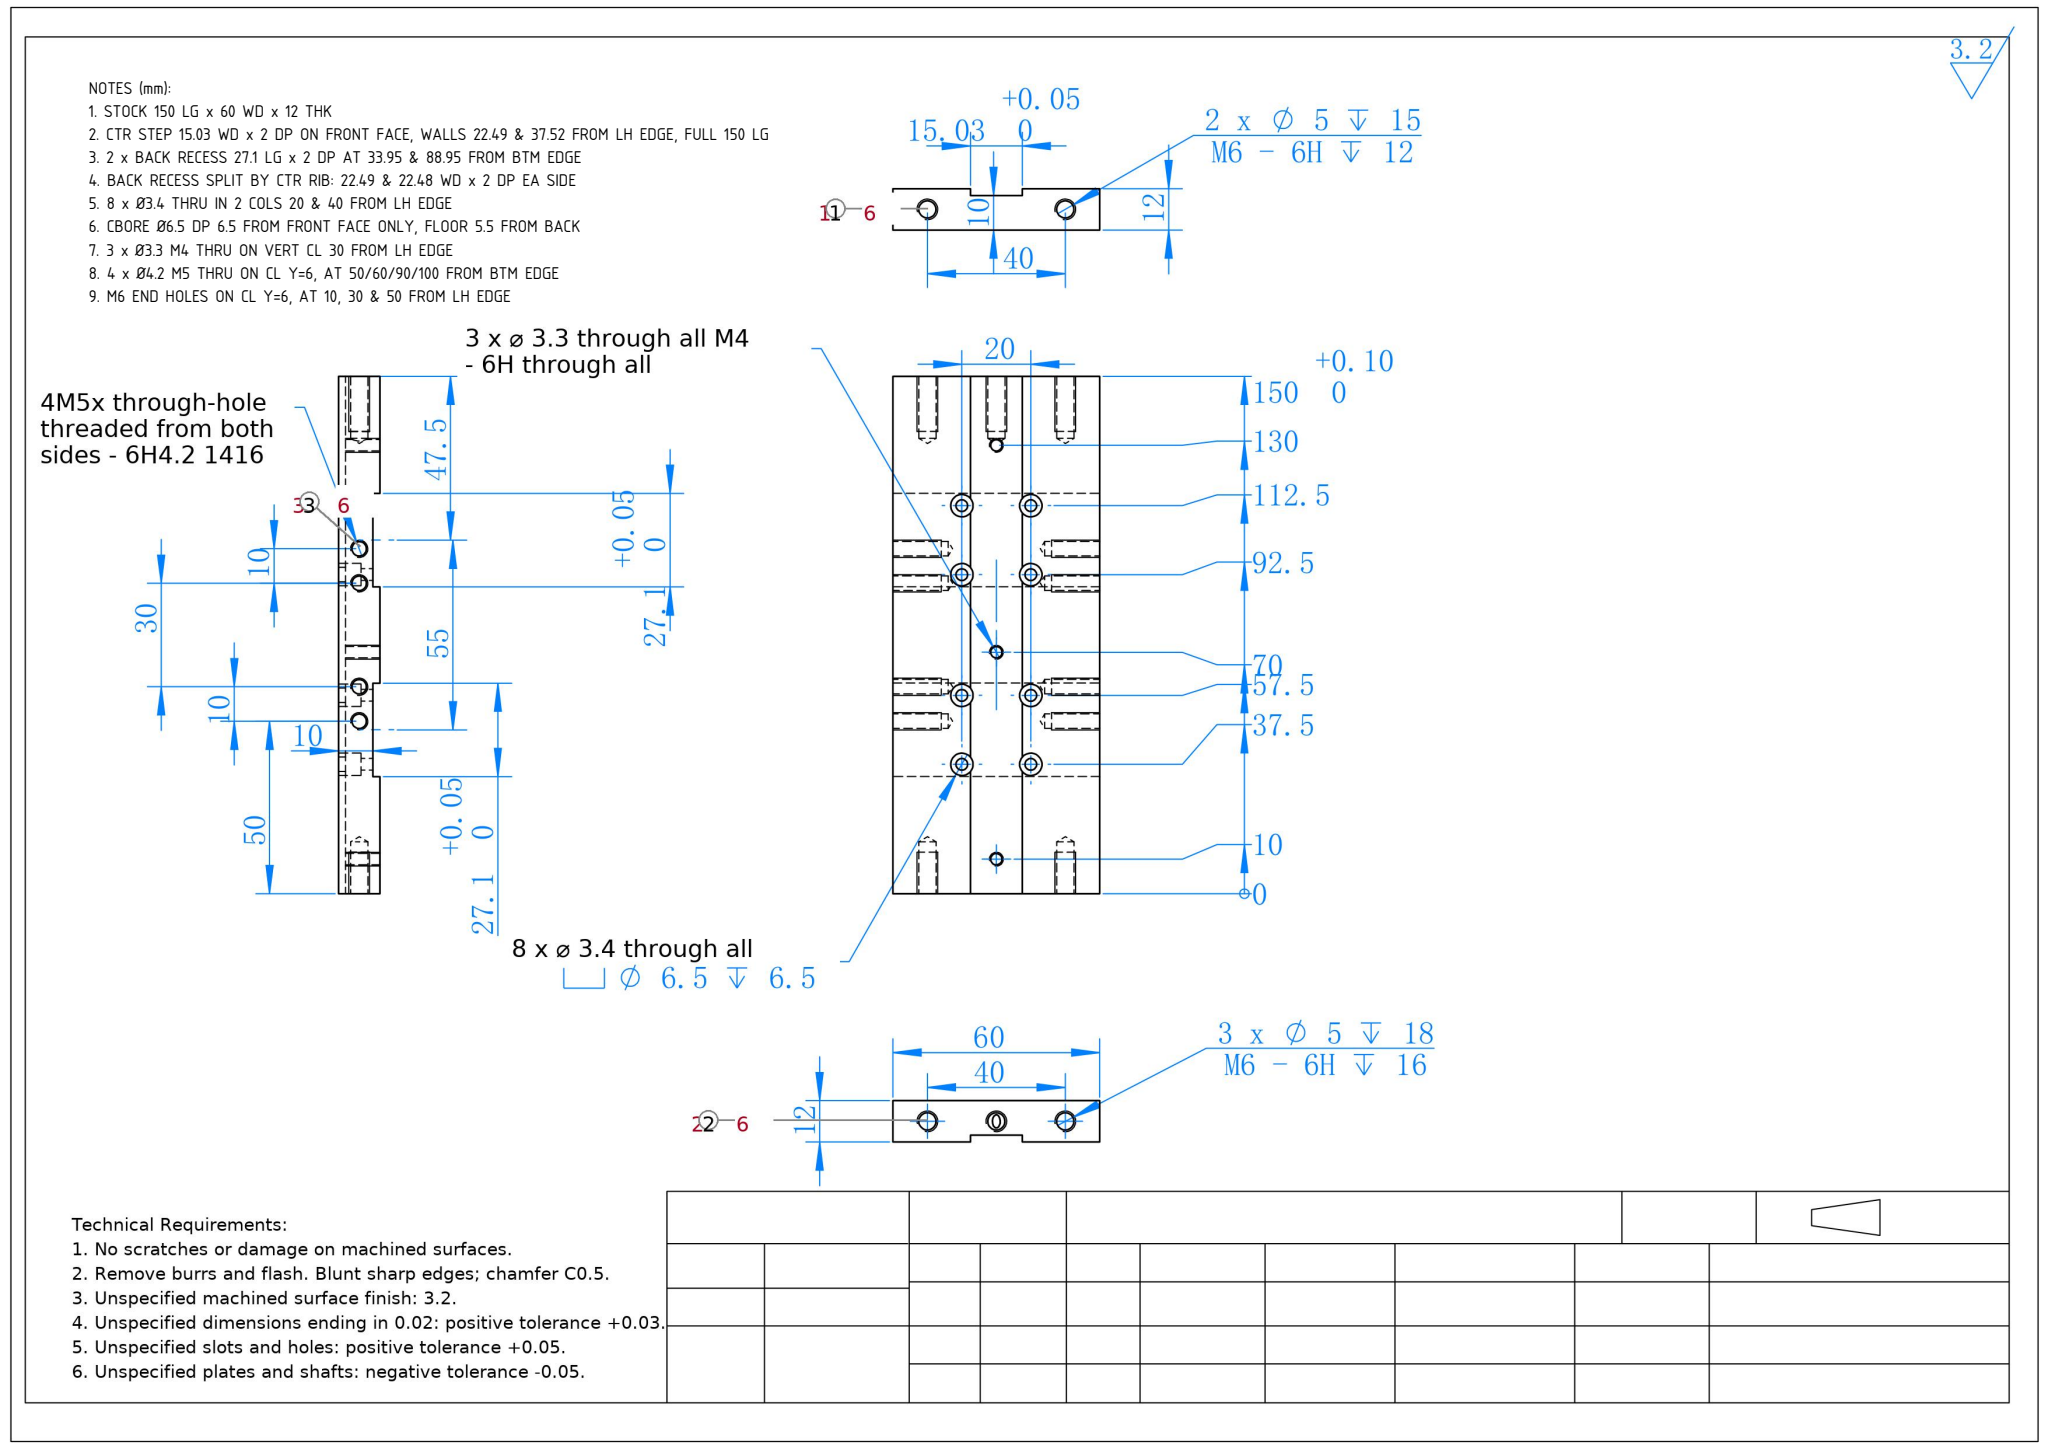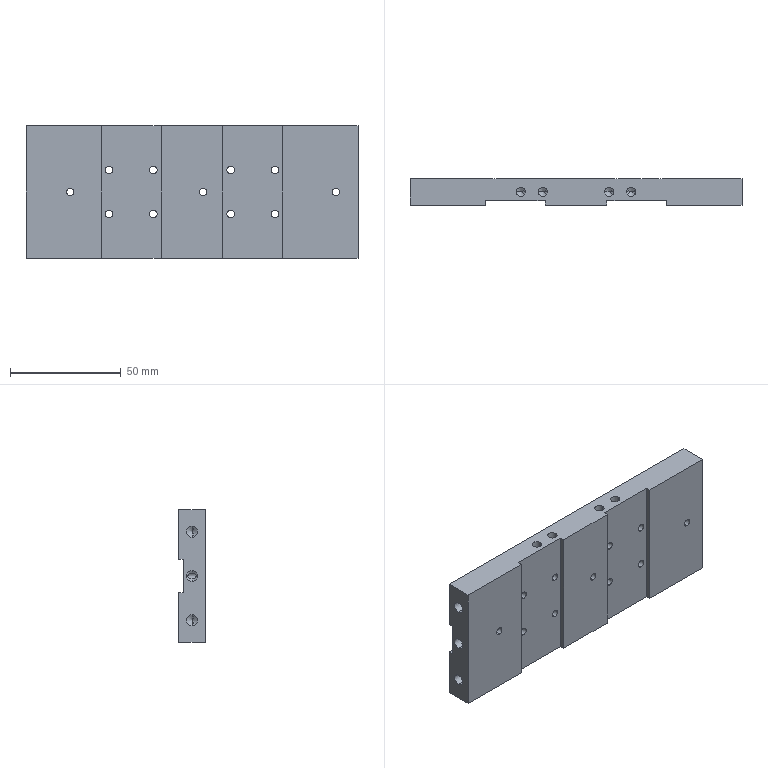Part | SolidWorks | mm | 1 solid | 124 faces | box 150 x 12 x 60 mm | volume 91270 mm3 | cylinder 64 | plane 34 | cone 26 | commonest cylinder face diameters 4.2 x16 6.5 x16 3.4 x16 5 x10 3.3 x6
Drawing notes:
STOCK 150 LG x 60 WD x 12 THK | from the solid: bbox_xyz 150.0 x 12.0 x 60.0
CTR STEP 15.03 WD x 2 DP ON FRONT FACE, WALLS 22.49 & 37.52 FROM LH EDGE, FULL 150 LG | from the solid: z-planes 22.49/37.52 (dif 15.03); y-plane 10.0 vs front face y=12.0
2 x BACK RECESS 27.1 LG x 2 DP AT 33.95 & 88.95 FROM BTM EDGE | from the solid: x-planes 33.95/61.05 and 88.95/116.05; y-plane 2.0 vs back face y=0
BACK RECESS SPLIT BY CTR RIB: 22.49 & 22.48 WD x 2 DP EA SIDE | from the solid: recess z 0-22.49 and 37.52-60.0, floor y=2.0
8 x Ø3.4 THRU IN 2 COLS 20 & 40 FROM LH EDGE | from the solid: Ø3.4 cyl axis y at z=20 and z=40, x=37.5/57.5/92.5/112.5
CBORE Ø6.5 DP 6.5 FROM FRONT FACE ONLY, FLOOR 5.5 FROM BACK | from the solid: Ø6.5 cyl axis y L=6.5; y-planes at 5.5 (8 off), part 12 thk
3 x Ø3.3 M4 THRU ON VERT CL 30 FROM LH EDGE | from the solid: Ø3.3 cyl axis y at z=30.0, x=20/80/140
4 x Ø4.2 M5 THRU ON CL Y=6, AT 50/60/90/100 FROM BTM EDGE | from the solid: Ø4.2 cyl axis z at x=50,60,90,100, y=6.0, L=16.0
M6 END HOLES ON CL Y=6, AT 10, 30 & 50 FROM LH EDGE | from the solid: Ø5 cyl axis x at z=10, 30, 50, y=6.0
build123d program:
from build123d import *

# Parameters (mm, degrees)
SKETCH1_W                                       = 150
SKETCH1_H                                       = 12
EXTRUDE1_DEPTH                                  = 30
SKETCH20_W                                      = 150
SKETCH20_H                                      = 15.03
CUT_EXTRUDE3_DEPTH                              = 2
SKETCH31_W                                      = 27.1
SKETCH31_H                                      = 60
CUT_EXTRUDE4_DEPTH                              = 2
M6_TAPPED_HOLE2_D                               = 5
M6_TAPPED_HOLE2_DEPTH                           = 18
M6_TAPPED_HOLE2_TIP                             = 1.502
M4_TAPPED_HOLE1_D                               = 3.3
M3_HEX_SOCKET_HEAD_CAP_SCREW_CBORE1_D           = 3.4
M3_HEX_SOCKET_HEAD_CAP_SCREW_CBORE1_CBORE_D     = 6.5
M3_HEX_SOCKET_HEAD_CAP_SCREW_CBORE1_CBORE_DEPTH = 6.5
M6_TAPPED_HOLE1_D                               = 5
M6_TAPPED_HOLE1_DEPTH                           = 15
M6_TAPPED_HOLE1_TIP                             = 1.502
M5_TAPPED_HOLE1_D                               = 4.2
M5_TAPPED_HOLE1_DEPTH                           = 16
M5_TAPPED_HOLE1_TIP                             = 1.262
M5_TAPPED_HOLE3_D                               = 4.2
M5_TAPPED_HOLE3_DEPTH                           = 16
M5_TAPPED_HOLE3_TIP                             = 1.262


with BuildPart() as part:
    # Sketch1 → Extrude1 (new, symmetric)
    with BuildSketch(Plane.XY):
        Rectangle(SKETCH1_W, SKETCH1_H)
    extrude(amount=EXTRUDE1_DEPTH, both=True)

    # Sketch20 → Cut-Extrude3 (cut)
    with BuildSketch(Plane(origin=(0, 6, 0), x_dir=(-1, 0, 0), z_dir=(0, 1, 0))):
        Rectangle(SKETCH20_W, SKETCH20_H)
    extrude(amount=-CUT_EXTRUDE3_DEPTH, mode=Mode.SUBTRACT)

    # Sketch31 → Cut-Extrude4 (cut)
    with BuildSketch(Plane(origin=(0, -6, 0), x_dir=(-1, 0, 0), z_dir=(0, -1, 0))):
        with Locations((27.5, 0)):
            Rectangle(SKETCH31_W, SKETCH31_H)
        with Locations((-27.5, 0)):
            Rectangle(SKETCH31_W, SKETCH31_H)
    extrude(amount=-CUT_EXTRUDE4_DEPTH, mode=Mode.SUBTRACT)

    # M6 Tapped Hole2
    with Locations(Plane.ZY.offset(75)):
        with Locations((-20, 0), (20, 0), (0, 0)):
            Hole(M6_TAPPED_HOLE2_D / 2, depth=M6_TAPPED_HOLE2_DEPTH)
            with Locations((0, 0, -(M6_TAPPED_HOLE2_DEPTH + M6_TAPPED_HOLE2_TIP / 2))):  # 118° drill point
                Cone(0, M6_TAPPED_HOLE2_D / 2, M6_TAPPED_HOLE2_TIP, mode=Mode.SUBTRACT)

    # M4 Tapped Hole1 (through all)
    with Locations(Plane(origin=(0, 6, 0), x_dir=(1, 0, 0), z_dir=(0, 1, 0))):
        with Locations((5, 0), (65, 0), (-55, 0)):
            Hole(M4_TAPPED_HOLE1_D / 2)

    # M3 Hex Socket Head Cap Screw CBORE1 (through all)
    with Locations(Plane(origin=(0, 6, 0), x_dir=(1, 0, 0), z_dir=(0, 1, 0))):
        with Locations((-37.5, 10), (-17.5, 10), (-37.5, -10), (-17.5, -10), (17.5, 10), (37.5, 10), (17.5, -10), (37.5, -10)):
            CounterBoreHole(M3_HEX_SOCKET_HEAD_CAP_SCREW_CBORE1_D / 2, M3_HEX_SOCKET_HEAD_CAP_SCREW_CBORE1_CBORE_D / 2, M3_HEX_SOCKET_HEAD_CAP_SCREW_CBORE1_CBORE_DEPTH)

    # M6 Tapped Hole1
    with Locations(Plane(origin=(75, 0, 0), x_dir=(0, 0, -1), z_dir=(1, 0, 0))):
        with Locations((-20, 0), (20, 0)):
            Hole(M6_TAPPED_HOLE1_D / 2, depth=M6_TAPPED_HOLE1_DEPTH)
            with Locations((0, 0, -(M6_TAPPED_HOLE1_DEPTH + M6_TAPPED_HOLE1_TIP / 2))):  # 118° drill point
                Cone(0, M6_TAPPED_HOLE1_D / 2, M6_TAPPED_HOLE1_TIP, mode=Mode.SUBTRACT)

    # M5 Tapped Hole1
    with Locations(Plane(origin=(0, 0, -30), x_dir=(1, 0, 0), z_dir=(0, 0, -1))):
        with Locations((-15, 0), (15, 0), (25, 0), (-25, 0)):
            Hole(M5_TAPPED_HOLE1_D / 2, depth=M5_TAPPED_HOLE1_DEPTH)
            with Locations((0, 0, -(M5_TAPPED_HOLE1_DEPTH + M5_TAPPED_HOLE1_TIP / 2))):  # 118° drill point
                Cone(0, M5_TAPPED_HOLE1_D / 2, M5_TAPPED_HOLE1_TIP, mode=Mode.SUBTRACT)

    # M5 Tapped Hole3
    with Locations(Plane.XY.offset(30)):
        with Locations((15, 0), (-15, 0), (-25, 0), (25, 0)):
            Hole(M5_TAPPED_HOLE3_D / 2, depth=M5_TAPPED_HOLE3_DEPTH)
            with Locations((0, 0, -(M5_TAPPED_HOLE3_DEPTH + M5_TAPPED_HOLE3_TIP / 2))):  # 118° drill point
                Cone(0, M5_TAPPED_HOLE3_D / 2, M5_TAPPED_HOLE3_TIP, mode=Mode.SUBTRACT)


solid = part.part